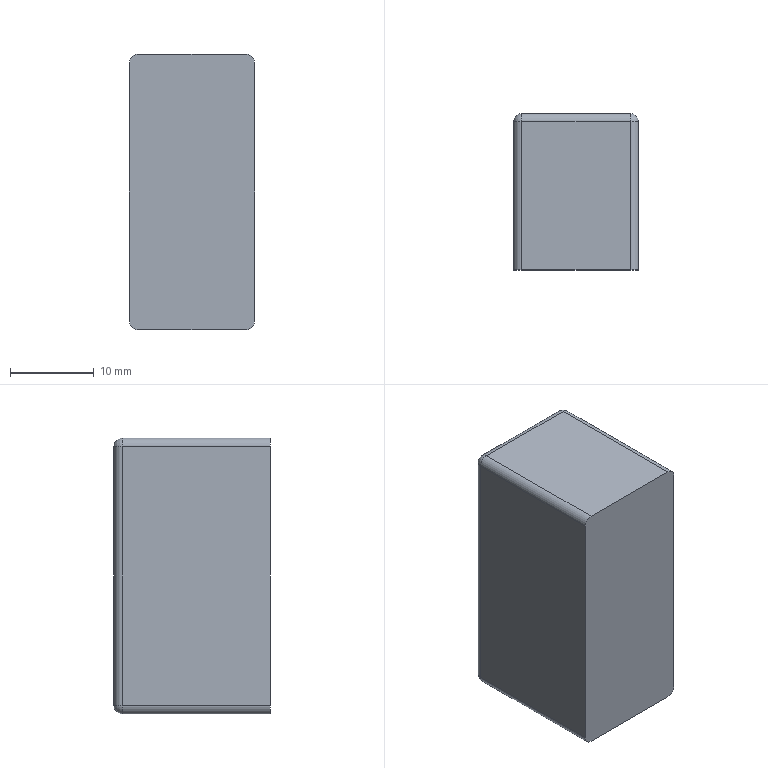Component | SolidWorks | StorageBox-1 | 1 solid | 23 faces | box 15 x 18.73 x 33 mm | volume 3493 mm3 | plane 11 | cylinder 8 | sphere 4 | commonest cylinder face diameters 2 x8
STEP:
#1=CARTESIAN_POINT('',(-0.8525,-3.531,8.395));
#2=VERTEX_POINT('',#1);
#3=CARTESIAN_POINT('',(-1.364,-3.531,8.395));
#4=VERTEX_POINT('',#3);
#5=CARTESIAN_POINT('',(-0.8131,-3.531,8.395));
#6=DIRECTION('',(-1.,-0.,0.));
#7=VECTOR('',#6,39.37);
#8=LINE('',#5,#7);
#9=EDGE_CURVE('',#2,#4,#8,.T.);
#10=ORIENTED_EDGE('',*,*,#9,.T.);
#11=CARTESIAN_POINT('',(-1.364,-4.229,8.395));
#12=VERTEX_POINT('',#11);
#13=CARTESIAN_POINT('',(-1.364,-4.229,8.395));
#14=DIRECTION('',(0.,-1.,0.));
#15=VECTOR('',#14,39.37);
#16=LINE('',#13,#15);
#17=EDGE_CURVE('',#4,#12,#16,.T.);
#18=ORIENTED_EDGE('',*,*,#17,.T.);
#19=CARTESIAN_POINT('',(-0.8525,-4.229,8.395));
#20=VERTEX_POINT('',#19);
#21=CARTESIAN_POINT('',(-0.8131,-4.229,8.395));
#22=DIRECTION('',(-1.,-0.,0.));
#23=VECTOR('',#22,39.37);
#24=LINE('',#21,#23);
#25=EDGE_CURVE('',#20,#12,#24,.T.);
#26=ORIENTED_EDGE('',*,*,#25,.F.);
#27=CARTESIAN_POINT('',(-0.8525,-4.229,8.395));
#28=DIRECTION('',(-0.,1.,-0.));
#29=VECTOR('',#28,39.37);
#30=LINE('',#27,#29);
#31=EDGE_CURVE('',#20,#2,#30,.T.);
#32=ORIENTED_EDGE('',*,*,#31,.T.);
#33=EDGE_LOOP('',(#10,#18,#26,#32));
#34=FACE_OUTER_BOUND('',#33,.T.);
#35=CARTESIAN_POINT('',(-0.8131,-4.229,8.395));
#36=DIRECTION('',(-0.,-0.,-1.));
#37=DIRECTION('',(-1.,-0.,0.));
#38=AXIS2_PLACEMENT_3D('',#35,#36,#37);
#39=PLANE('',#38);
#40=ADVANCED_FACE('',(#34),#39,.F.);
#41=CARTESIAN_POINT('',(-0.8525,-4.229,7.096));
#42=VERTEX_POINT('',#41);
#43=CARTESIAN_POINT('',(-1.364,-4.229,7.096));
#44=VERTEX_POINT('',#43);
#45=CARTESIAN_POINT('',(-0.8131,-4.229,7.096));
#46=DIRECTION('',(-1.,-0.,0.));
#47=VECTOR('',#46,39.37);
#48=LINE('',#45,#47);
#49=EDGE_CURVE('',#42,#44,#48,.T.);
#50=ORIENTED_EDGE('',*,*,#49,.F.);
#51=CARTESIAN_POINT('',(-0.8131,-4.229,7.136));
#52=VERTEX_POINT('',#51);
#53=CARTESIAN_POINT('',(-0.8525,-4.229,7.136));
#54=DIRECTION('',(0.,-1.,0.));
#55=DIRECTION('',(1.,0.,0.));
#56=AXIS2_PLACEMENT_3D('',#53,#54,#55);
#57=CIRCLE('',#56,0.03937);
#58=EDGE_CURVE('',#42,#52,#57,.T.);
#59=ORIENTED_EDGE('',*,*,#58,.T.);
#60=CARTESIAN_POINT('',(-0.8131,-4.229,8.356));
#61=VERTEX_POINT('',#60);
#62=CARTESIAN_POINT('',(-0.8131,-4.229,8.395));
#63=DIRECTION('',(-0.,-0.,-1.));
#64=VECTOR('',#63,39.37);
#65=LINE('',#62,#64);
#66=EDGE_CURVE('',#61,#52,#65,.T.);
#67=ORIENTED_EDGE('',*,*,#66,.F.);
#68=CARTESIAN_POINT('',(-0.8525,-4.229,8.356));
#69=DIRECTION('',(0.,-1.,0.));
#70=DIRECTION('',(1.,0.,0.));
#71=AXIS2_PLACEMENT_3D('',#68,#69,#70);
#72=CIRCLE('',#71,0.03937);
#73=EDGE_CURVE('',#61,#20,#72,.T.);
#74=ORIENTED_EDGE('',*,*,#73,.T.);
#75=ORIENTED_EDGE('',*,*,#25,.T.);
#76=CARTESIAN_POINT('',(-1.404,-4.229,8.356));
#77=VERTEX_POINT('',#76);
#78=CARTESIAN_POINT('',(-1.364,-4.229,8.356));
#79=DIRECTION('',(0.,-1.,0.));
#80=DIRECTION('',(1.,0.,0.));
#81=AXIS2_PLACEMENT_3D('',#78,#79,#80);
#82=CIRCLE('',#81,0.03937);
#83=EDGE_CURVE('',#12,#77,#82,.T.);
#84=ORIENTED_EDGE('',*,*,#83,.T.);
#85=CARTESIAN_POINT('',(-1.404,-4.229,7.136));
#86=VERTEX_POINT('',#85);
#87=CARTESIAN_POINT('',(-1.404,-4.229,8.395));
#88=DIRECTION('',(-0.,-0.,-1.));
#89=VECTOR('',#88,39.37);
#90=LINE('',#87,#89);
#91=EDGE_CURVE('',#77,#86,#90,.T.);
#92=ORIENTED_EDGE('',*,*,#91,.T.);
#93=CARTESIAN_POINT('',(-1.364,-4.229,7.136));
#94=DIRECTION('',(0.,-1.,0.));
#95=DIRECTION('',(1.,0.,0.));
#96=AXIS2_PLACEMENT_3D('',#93,#94,#95);
#97=CIRCLE('',#96,0.03937);
#98=EDGE_CURVE('',#86,#44,#97,.T.);
#99=ORIENTED_EDGE('',*,*,#98,.T.);
#100=EDGE_LOOP('',(#50,#59,#67,#74,#75,#84,#92,#99));
#101=FACE_OUTER_BOUND('',#100,.T.);
#102=CARTESIAN_POINT('',(-0.8131,-4.229,8.395));
#103=DIRECTION('',(-0.,1.,-0.));
#104=DIRECTION('',(1.,0.,-0.));
#105=AXIS2_PLACEMENT_3D('',#102,#103,#104);
#106=PLANE('',#105);
#107=ADVANCED_FACE('',(#101),#106,.F.);
#108=CARTESIAN_POINT('',(-1.364,-3.531,7.096));
#109=VERTEX_POINT('',#108);
#110=CARTESIAN_POINT('',(-0.8525,-3.531,7.096));
#111=VERTEX_POINT('',#110);
#112=CARTESIAN_POINT('',(-0.8131,-3.531,7.096));
#113=DIRECTION('',(1.,0.,-0.));
#114=VECTOR('',#113,39.37);
#115=LINE('',#112,#114);
#116=EDGE_CURVE('',#109,#111,#115,.T.);
#117=ORIENTED_EDGE('',*,*,#116,.T.);
#118=CARTESIAN_POINT('',(-0.8525,-4.229,7.096));
#119=DIRECTION('',(0.,-1.,0.));
#120=VECTOR('',#119,39.37);
#121=LINE('',#118,#120);
#122=EDGE_CURVE('',#111,#42,#121,.T.);
#123=ORIENTED_EDGE('',*,*,#122,.T.);
#124=ORIENTED_EDGE('',*,*,#49,.T.);
#125=CARTESIAN_POINT('',(-1.364,-3.531,7.096));
#126=DIRECTION('',(-0.,1.,-0.));
#127=VECTOR('',#126,39.37);
#128=LINE('',#125,#127);
#129=EDGE_CURVE('',#44,#109,#128,.T.);
#130=ORIENTED_EDGE('',*,*,#129,.T.);
#131=EDGE_LOOP('',(#117,#123,#124,#130));
#132=FACE_OUTER_BOUND('',#131,.T.);
#133=CARTESIAN_POINT('',(-0.8131,-4.229,7.096));
#134=DIRECTION('',(0.,0.,1.));
#135=DIRECTION('',(1.,0.,-0.));
#136=AXIS2_PLACEMENT_3D('',#133,#134,#135);
#137=PLANE('',#136);
#138=ADVANCED_FACE('',(#132),#137,.F.);
#139=CARTESIAN_POINT('',(-1.364,-3.492,8.356));
#140=VERTEX_POINT('',#139);
#141=CARTESIAN_POINT('',(-0.8525,-3.492,8.356));
#142=VERTEX_POINT('',#141);
#143=CARTESIAN_POINT('',(-0.8131,-3.492,8.356));
#144=DIRECTION('',(1.,0.,-0.));
#145=VECTOR('',#144,39.37);
#146=LINE('',#143,#145);
#147=EDGE_CURVE('',#140,#142,#146,.T.);
#148=ORIENTED_EDGE('',*,*,#147,.T.);
#149=CARTESIAN_POINT('',(-0.8525,-3.492,7.136));
#150=VERTEX_POINT('',#149);
#151=CARTESIAN_POINT('',(-0.8525,-3.492,8.395));
#152=DIRECTION('',(-0.,-0.,-1.));
#153=VECTOR('',#152,39.37);
#154=LINE('',#151,#153);
#155=EDGE_CURVE('',#142,#150,#154,.T.);
#156=ORIENTED_EDGE('',*,*,#155,.T.);
#157=CARTESIAN_POINT('',(-1.364,-3.492,7.136));
#158=VERTEX_POINT('',#157);
#159=CARTESIAN_POINT('',(-0.8131,-3.492,7.136));
#160=DIRECTION('',(-1.,-0.,0.));
#161=VECTOR('',#160,39.37);
#162=LINE('',#159,#161);
#163=EDGE_CURVE('',#150,#158,#162,.T.);
#164=ORIENTED_EDGE('',*,*,#163,.T.);
#165=CARTESIAN_POINT('',(-1.364,-3.492,8.395));
#166=DIRECTION('',(0.,0.,1.));
#167=VECTOR('',#166,39.37);
#168=LINE('',#165,#167);
#169=EDGE_CURVE('',#158,#140,#168,.T.);
#170=ORIENTED_EDGE('',*,*,#169,.T.);
#171=EDGE_LOOP('',(#148,#156,#164,#170));
#172=FACE_OUTER_BOUND('',#171,.T.);
#173=CARTESIAN_POINT('',(-1.325,-3.492,7.175));
#174=VERTEX_POINT('',#173);
#175=CARTESIAN_POINT('',(-1.325,-3.492,8.317));
#176=VERTEX_POINT('',#175);
#177=CARTESIAN_POINT('',(-1.325,-3.492,7.175));
#178=DIRECTION('',(0.,0.,1.));
#179=VECTOR('',#178,39.37);
#180=LINE('',#177,#179);
#181=EDGE_CURVE('',#174,#176,#180,.T.);
#182=ORIENTED_EDGE('',*,*,#181,.F.);
#183=CARTESIAN_POINT('',(-0.8919,-3.492,7.175));
#184=VERTEX_POINT('',#183);
#185=CARTESIAN_POINT('',(-0.8919,-3.492,7.175));
#186=DIRECTION('',(-1.,-0.,0.));
#187=VECTOR('',#186,39.37);
#188=LINE('',#185,#187);
#189=EDGE_CURVE('',#184,#174,#188,.T.);
#190=ORIENTED_EDGE('',*,*,#189,.F.);
#191=CARTESIAN_POINT('',(-0.8919,-3.492,8.317));
#192=VERTEX_POINT('',#191);
#193=CARTESIAN_POINT('',(-0.8919,-3.492,8.317));
#194=DIRECTION('',(-0.,-0.,-1.));
#195=VECTOR('',#194,39.37);
#196=LINE('',#193,#195);
#197=EDGE_CURVE('',#192,#184,#196,.T.);
#198=ORIENTED_EDGE('',*,*,#197,.F.);
#199=CARTESIAN_POINT('',(-1.325,-3.492,8.317));
#200=DIRECTION('',(1.,0.,-0.));
#201=VECTOR('',#200,39.37);
#202=LINE('',#199,#201);
#203=EDGE_CURVE('',#176,#192,#202,.T.);
#204=ORIENTED_EDGE('',*,*,#203,.F.);
#205=EDGE_LOOP('',(#182,#190,#198,#204));
#206=FACE_BOUND('',#205,.T.);
#207=CARTESIAN_POINT('',(-0.8131,-3.492,8.395));
#208=DIRECTION('',(0.,-1.,0.));
#209=DIRECTION('',(-1.,-0.,0.));
#210=AXIS2_PLACEMENT_3D('',#207,#208,#209);
#211=PLANE('',#210);
#212=ADVANCED_FACE('',(#172,#206),#211,.F.);
#213=ORIENTED_EDGE('',*,*,#66,.T.);
#214=CARTESIAN_POINT('',(-0.8131,-3.531,7.136));
#215=VERTEX_POINT('',#214);
#216=CARTESIAN_POINT('',(-0.8131,-4.229,7.136));
#217=DIRECTION('',(-0.,1.,-0.));
#218=VECTOR('',#217,39.37);
#219=LINE('',#216,#218);
#220=EDGE_CURVE('',#52,#215,#219,.T.);
#221=ORIENTED_EDGE('',*,*,#220,.T.);
#222=CARTESIAN_POINT('',(-0.8131,-3.531,8.356));
#223=VERTEX_POINT('',#222);
#224=CARTESIAN_POINT('',(-0.8131,-3.531,8.395));
#225=DIRECTION('',(0.,0.,1.));
#226=VECTOR('',#225,39.37);
#227=LINE('',#224,#226);
#228=EDGE_CURVE('',#215,#223,#227,.T.);
#229=ORIENTED_EDGE('',*,*,#228,.T.);
#230=CARTESIAN_POINT('',(-0.8131,-4.229,8.356));
#231=DIRECTION('',(0.,-1.,0.));
#232=VECTOR('',#231,39.37);
#233=LINE('',#230,#232);
#234=EDGE_CURVE('',#223,#61,#233,.T.);
#235=ORIENTED_EDGE('',*,*,#234,.T.);
#236=EDGE_LOOP('',(#213,#221,#229,#235));
#237=FACE_OUTER_BOUND('',#236,.T.);
#238=CARTESIAN_POINT('',(-0.8131,-4.229,8.395));
#239=DIRECTION('',(-1.,-0.,0.));
#240=DIRECTION('',(0.,0.,1.));
#241=AXIS2_PLACEMENT_3D('',#238,#239,#240);
#242=PLANE('',#241);
#243=ADVANCED_FACE('',(#237),#242,.F.);
#244=CARTESIAN_POINT('',(-1.404,-3.531,8.356));
#245=VERTEX_POINT('',#244);
#246=CARTESIAN_POINT('',(-1.404,-3.531,7.136));
#247=VERTEX_POINT('',#246);
#248=CARTESIAN_POINT('',(-1.404,-3.531,7.096));
#249=DIRECTION('',(-0.,-0.,-1.));
#250=VECTOR('',#249,39.37);
#251=LINE('',#248,#250);
#252=EDGE_CURVE('',#245,#247,#251,.T.);
#253=ORIENTED_EDGE('',*,*,#252,.T.);
#254=CARTESIAN_POINT('',(-1.404,-4.229,7.136));
#255=DIRECTION('',(0.,-1.,0.));
#256=VECTOR('',#255,39.37);
#257=LINE('',#254,#256);
#258=EDGE_CURVE('',#247,#86,#257,.T.);
#259=ORIENTED_EDGE('',*,*,#258,.T.);
#260=ORIENTED_EDGE('',*,*,#91,.F.);
#261=CARTESIAN_POINT('',(-1.404,-3.531,8.356));
#262=DIRECTION('',(-0.,1.,-0.));
#263=VECTOR('',#262,39.37);
#264=LINE('',#261,#263);
#265=EDGE_CURVE('',#77,#245,#264,.T.);
#266=ORIENTED_EDGE('',*,*,#265,.T.);
#267=EDGE_LOOP('',(#253,#259,#260,#266));
#268=FACE_OUTER_BOUND('',#267,.T.);
#269=CARTESIAN_POINT('',(-1.404,-4.229,8.395));
#270=DIRECTION('',(-1.,-0.,0.));
#271=DIRECTION('',(0.,0.,1.));
#272=AXIS2_PLACEMENT_3D('',#269,#270,#271);
#273=PLANE('',#272);
#274=ADVANCED_FACE('',(#268),#273,.T.);
#275=ORIENTED_EDGE('',*,*,#189,.T.);
#276=CARTESIAN_POINT('',(-1.325,-4.2,7.175));
#277=VERTEX_POINT('',#276);
#278=CARTESIAN_POINT('',(-1.325,-4.2,7.175));
#279=DIRECTION('',(-0.,1.,-0.));
#280=VECTOR('',#279,39.37);
#281=LINE('',#278,#280);
#282=EDGE_CURVE('',#277,#174,#281,.T.);
#283=ORIENTED_EDGE('',*,*,#282,.F.);
#284=CARTESIAN_POINT('',(-0.8919,-4.2,7.175));
#285=VERTEX_POINT('',#284);
#286=CARTESIAN_POINT('',(-0.8919,-4.2,7.175));
#287=DIRECTION('',(-1.,-0.,0.));
#288=VECTOR('',#287,39.37);
#289=LINE('',#286,#288);
#290=EDGE_CURVE('',#285,#277,#289,.T.);
#291=ORIENTED_EDGE('',*,*,#290,.F.);
#292=CARTESIAN_POINT('',(-0.8919,-4.2,7.175));
#293=DIRECTION('',(-0.,1.,-0.));
#294=VECTOR('',#293,39.37);
#295=LINE('',#292,#294);
#296=EDGE_CURVE('',#285,#184,#295,.T.);
#297=ORIENTED_EDGE('',*,*,#296,.T.);
#298=EDGE_LOOP('',(#275,#283,#291,#297));
#299=FACE_OUTER_BOUND('',#298,.T.);
#300=CARTESIAN_POINT('',(-0.8919,-4.2,7.175));
#301=DIRECTION('',(-0.,-0.,-1.));
#302=DIRECTION('',(-1.,-0.,0.));
#303=AXIS2_PLACEMENT_3D('',#300,#301,#302);
#304=PLANE('',#303);
#305=ADVANCED_FACE('',(#299),#304,.F.);
#306=ORIENTED_EDGE('',*,*,#197,.T.);
#307=ORIENTED_EDGE('',*,*,#296,.F.);
#308=CARTESIAN_POINT('',(-0.8919,-4.2,8.317));
#309=VERTEX_POINT('',#308);
#310=CARTESIAN_POINT('',(-0.8919,-4.2,8.317));
#311=DIRECTION('',(-0.,-0.,-1.));
#312=VECTOR('',#311,39.37);
#313=LINE('',#310,#312);
#314=EDGE_CURVE('',#309,#285,#313,.T.);
#315=ORIENTED_EDGE('',*,*,#314,.F.);
#316=CARTESIAN_POINT('',(-0.8919,-4.2,8.317));
#317=DIRECTION('',(-0.,1.,-0.));
#318=VECTOR('',#317,39.37);
#319=LINE('',#316,#318);
#320=EDGE_CURVE('',#309,#192,#319,.T.);
#321=ORIENTED_EDGE('',*,*,#320,.T.);
#322=EDGE_LOOP('',(#306,#307,#315,#321));
#323=FACE_OUTER_BOUND('',#322,.T.);
#324=CARTESIAN_POINT('',(-0.8919,-4.2,8.317));
#325=DIRECTION('',(1.,0.,-0.));
#326=DIRECTION('',(-0.,-0.,-1.));
#327=AXIS2_PLACEMENT_3D('',#324,#325,#326);
#328=PLANE('',#327);
#329=ADVANCED_FACE('',(#323),#328,.F.);
#330=ORIENTED_EDGE('',*,*,#203,.T.);
#331=ORIENTED_EDGE('',*,*,#320,.F.);
#332=CARTESIAN_POINT('',(-1.325,-4.2,8.317));
#333=VERTEX_POINT('',#332);
#334=CARTESIAN_POINT('',(-1.325,-4.2,8.317));
#335=DIRECTION('',(1.,0.,-0.));
#336=VECTOR('',#335,39.37);
#337=LINE('',#334,#336);
#338=EDGE_CURVE('',#333,#309,#337,.T.);
#339=ORIENTED_EDGE('',*,*,#338,.F.);
#340=CARTESIAN_POINT('',(-1.325,-4.2,8.317));
#341=DIRECTION('',(-0.,1.,-0.));
#342=VECTOR('',#341,39.37);
#343=LINE('',#340,#342);
#344=EDGE_CURVE('',#333,#176,#343,.T.);
#345=ORIENTED_EDGE('',*,*,#344,.T.);
#346=EDGE_LOOP('',(#330,#331,#339,#345));
#347=FACE_OUTER_BOUND('',#346,.T.);
#348=CARTESIAN_POINT('',(-1.325,-4.2,8.317));
#349=DIRECTION('',(0.,0.,1.));
#350=DIRECTION('',(1.,0.,-0.));
#351=AXIS2_PLACEMENT_3D('',#348,#349,#350);
#352=PLANE('',#351);
#353=ADVANCED_FACE('',(#347),#352,.F.);
#354=ORIENTED_EDGE('',*,*,#181,.T.);
#355=ORIENTED_EDGE('',*,*,#344,.F.);
#356=CARTESIAN_POINT('',(-1.325,-4.2,7.175));
#357=DIRECTION('',(0.,0.,1.));
#358=VECTOR('',#357,39.37);
#359=LINE('',#356,#358);
#360=EDGE_CURVE('',#277,#333,#359,.T.);
#361=ORIENTED_EDGE('',*,*,#360,.F.);
#362=ORIENTED_EDGE('',*,*,#282,.T.);
#363=EDGE_LOOP('',(#354,#355,#361,#362));
#364=FACE_OUTER_BOUND('',#363,.T.);
#365=CARTESIAN_POINT('',(-1.325,-4.2,7.175));
#366=DIRECTION('',(-1.,-0.,0.));
#367=DIRECTION('',(0.,0.,1.));
#368=AXIS2_PLACEMENT_3D('',#365,#366,#367);
#369=PLANE('',#368);
#370=ADVANCED_FACE('',(#364),#369,.F.);
#371=ORIENTED_EDGE('',*,*,#290,.T.);
#372=ORIENTED_EDGE('',*,*,#360,.T.);
#373=ORIENTED_EDGE('',*,*,#338,.T.);
#374=ORIENTED_EDGE('',*,*,#314,.T.);
#375=EDGE_LOOP('',(#371,#372,#373,#374));
#376=FACE_OUTER_BOUND('',#375,.T.);
#377=CARTESIAN_POINT('',(-1.404,-4.2,8.395));
#378=DIRECTION('',(-0.,1.,-0.));
#379=DIRECTION('',(1.,0.,-0.));
#380=AXIS2_PLACEMENT_3D('',#377,#378,#379);
#381=PLANE('',#380);
#382=ADVANCED_FACE('',(#376),#381,.T.);
#383=ORIENTED_EDGE('',*,*,#169,.F.);
#384=CARTESIAN_POINT('',(-1.364,-3.531,7.136));
#385=DIRECTION('',(0.,0.,1.));
#386=DIRECTION('',(-1.,0.,0.));
#387=AXIS2_PLACEMENT_3D('',#384,#385,#386);
#388=CIRCLE('',#387,0.03937);
#389=EDGE_CURVE('',#158,#247,#388,.T.);
#390=ORIENTED_EDGE('',*,*,#389,.T.);
#391=ORIENTED_EDGE('',*,*,#252,.F.);
#392=CARTESIAN_POINT('',(-1.364,-3.531,8.356));
#393=DIRECTION('',(-0.,-0.,-1.));
#394=DIRECTION('',(-1.,0.,0.));
#395=AXIS2_PLACEMENT_3D('',#392,#393,#394);
#396=CIRCLE('',#395,0.03937);
#397=EDGE_CURVE('',#245,#140,#396,.T.);
#398=ORIENTED_EDGE('',*,*,#397,.T.);
#399=EDGE_LOOP('',(#383,#390,#391,#398));
#400=FACE_OUTER_BOUND('',#399,.T.);
#401=CARTESIAN_POINT('',(-1.364,-3.531,8.395));
#402=DIRECTION('',(-0.,-0.,-1.));
#403=DIRECTION('',(-1.,0.,0.));
#404=AXIS2_PLACEMENT_3D('',#401,#402,#403);
#405=CYLINDRICAL_SURFACE('',#404,0.03937);
#406=ADVANCED_FACE('',(#400),#405,.T.);
#407=ORIENTED_EDGE('',*,*,#163,.F.);
#408=CARTESIAN_POINT('',(-0.8525,-3.531,7.136));
#409=DIRECTION('',(-1.,-0.,0.));
#410=DIRECTION('',(0.,0.,1.));
#411=AXIS2_PLACEMENT_3D('',#408,#409,#410);
#412=CIRCLE('',#411,0.03937);
#413=EDGE_CURVE('',#150,#111,#412,.T.);
#414=ORIENTED_EDGE('',*,*,#413,.T.);
#415=ORIENTED_EDGE('',*,*,#116,.F.);
#416=CARTESIAN_POINT('',(-1.364,-3.531,7.136));
#417=DIRECTION('',(1.,0.,-0.));
#418=DIRECTION('',(0.,0.,1.));
#419=AXIS2_PLACEMENT_3D('',#416,#417,#418);
#420=CIRCLE('',#419,0.03937);
#421=EDGE_CURVE('',#109,#158,#420,.T.);
#422=ORIENTED_EDGE('',*,*,#421,.T.);
#423=EDGE_LOOP('',(#407,#414,#415,#422));
#424=FACE_OUTER_BOUND('',#423,.T.);
#425=CARTESIAN_POINT('',(-0.8131,-3.531,7.136));
#426=DIRECTION('',(-1.,-0.,0.));
#427=DIRECTION('',(0.,0.,1.));
#428=AXIS2_PLACEMENT_3D('',#425,#426,#427);
#429=CYLINDRICAL_SURFACE('',#428,0.03937);
#430=ADVANCED_FACE('',(#424),#429,.T.);
#431=ORIENTED_EDGE('',*,*,#147,.F.);
#432=CARTESIAN_POINT('',(-1.364,-3.531,8.356));
#433=DIRECTION('',(1.,0.,-0.));
#434=DIRECTION('',(0.,0.,1.));
#435=AXIS2_PLACEMENT_3D('',#432,#433,#434);
#436=CIRCLE('',#435,0.03937);
#437=EDGE_CURVE('',#140,#4,#436,.T.);
#438=ORIENTED_EDGE('',*,*,#437,.T.);
#439=ORIENTED_EDGE('',*,*,#9,.F.);
#440=CARTESIAN_POINT('',(-0.8525,-3.531,8.356));
#441=DIRECTION('',(-1.,-0.,0.));
#442=DIRECTION('',(0.,0.,1.));
#443=AXIS2_PLACEMENT_3D('',#440,#441,#442);
#444=CIRCLE('',#443,0.03937);
#445=EDGE_CURVE('',#2,#142,#444,.T.);
#446=ORIENTED_EDGE('',*,*,#445,.T.);
#447=EDGE_LOOP('',(#431,#438,#439,#446));
#448=FACE_OUTER_BOUND('',#447,.T.);
#449=CARTESIAN_POINT('',(-0.8131,-3.531,8.356));
#450=DIRECTION('',(-1.,-0.,0.));
#451=DIRECTION('',(0.,0.,1.));
#452=AXIS2_PLACEMENT_3D('',#449,#450,#451);
#453=CYLINDRICAL_SURFACE('',#452,0.03937);
#454=ADVANCED_FACE('',(#448),#453,.T.);
#455=ORIENTED_EDGE('',*,*,#228,.F.);
#456=CARTESIAN_POINT('',(-0.8525,-3.531,7.136));
#457=DIRECTION('',(0.,0.,1.));
#458=DIRECTION('',(1.,0.,0.));
#459=AXIS2_PLACEMENT_3D('',#456,#457,#458);
#460=CIRCLE('',#459,0.03937);
#461=EDGE_CURVE('',#215,#150,#460,.T.);
#462=ORIENTED_EDGE('',*,*,#461,.T.);
#463=ORIENTED_EDGE('',*,*,#155,.F.);
#464=CARTESIAN_POINT('',(-0.8525,-3.531,8.356));
#465=DIRECTION('',(-0.,-0.,-1.));
#466=DIRECTION('',(1.,0.,0.));
#467=AXIS2_PLACEMENT_3D('',#464,#465,#466);
#468=CIRCLE('',#467,0.03937);
#469=EDGE_CURVE('',#142,#223,#468,.T.);
#470=ORIENTED_EDGE('',*,*,#469,.T.);
#471=EDGE_LOOP('',(#455,#462,#463,#470));
#472=FACE_OUTER_BOUND('',#471,.T.);
#473=CARTESIAN_POINT('',(-0.8525,-3.531,8.395));
#474=DIRECTION('',(0.,0.,1.));
#475=DIRECTION('',(1.,0.,0.));
#476=AXIS2_PLACEMENT_3D('',#473,#474,#475);
#477=CYLINDRICAL_SURFACE('',#476,0.03937);
#478=ADVANCED_FACE('',(#472),#477,.T.);
#479=ORIENTED_EDGE('',*,*,#58,.F.);
#480=ORIENTED_EDGE('',*,*,#122,.F.);
#481=CARTESIAN_POINT('',(-0.8525,-3.531,7.136));
#482=DIRECTION('',(-0.,1.,-0.));
#483=DIRECTION('',(1.,0.,0.));
#484=AXIS2_PLACEMENT_3D('',#481,#482,#483);
#485=CIRCLE('',#484,0.03937);
#486=EDGE_CURVE('',#215,#111,#485,.T.);
#487=ORIENTED_EDGE('',*,*,#486,.F.);
#488=ORIENTED_EDGE('',*,*,#220,.F.);
#489=EDGE_LOOP('',(#479,#480,#487,#488));
#490=FACE_OUTER_BOUND('',#489,.T.);
#491=CARTESIAN_POINT('',(-0.8525,-4.229,7.136));
#492=DIRECTION('',(-0.,1.,-0.));
#493=DIRECTION('',(1.,0.,0.));
#494=AXIS2_PLACEMENT_3D('',#491,#492,#493);
#495=CYLINDRICAL_SURFACE('',#494,0.03937);
#496=ADVANCED_FACE('',(#490),#495,.T.);
#497=ORIENTED_EDGE('',*,*,#486,.T.);
#498=ORIENTED_EDGE('',*,*,#413,.F.);
#499=ORIENTED_EDGE('',*,*,#461,.F.);
#500=EDGE_LOOP('',(#497,#498,#499));
#501=FACE_OUTER_BOUND('',#500,.T.);
#502=CARTESIAN_POINT('',(-0.8525,-3.531,7.136));
#503=DIRECTION('',(-0.,1.,0.));
#504=DIRECTION('',(0.,0.,-1.));
#505=AXIS2_PLACEMENT_3D('',#502,#503,#504);
#506=SPHERICAL_SURFACE('',#505,0.03937);
#507=ADVANCED_FACE('',(#501),#506,.T.);
#508=ORIENTED_EDGE('',*,*,#98,.F.);
#509=ORIENTED_EDGE('',*,*,#258,.F.);
#510=CARTESIAN_POINT('',(-1.364,-3.531,7.136));
#511=DIRECTION('',(-0.,1.,-0.));
#512=DIRECTION('',(1.,0.,0.));
#513=AXIS2_PLACEMENT_3D('',#510,#511,#512);
#514=CIRCLE('',#513,0.03937);
#515=EDGE_CURVE('',#109,#247,#514,.T.);
#516=ORIENTED_EDGE('',*,*,#515,.F.);
#517=ORIENTED_EDGE('',*,*,#129,.F.);
#518=EDGE_LOOP('',(#508,#509,#516,#517));
#519=FACE_OUTER_BOUND('',#518,.T.);
#520=CARTESIAN_POINT('',(-1.364,-4.229,7.136));
#521=DIRECTION('',(0.,-1.,0.));
#522=DIRECTION('',(-1.,0.,0.));
#523=AXIS2_PLACEMENT_3D('',#520,#521,#522);
#524=CYLINDRICAL_SURFACE('',#523,0.03937);
#525=ADVANCED_FACE('',(#519),#524,.T.);
#526=ORIENTED_EDGE('',*,*,#515,.T.);
#527=ORIENTED_EDGE('',*,*,#389,.F.);
#528=ORIENTED_EDGE('',*,*,#421,.F.);
#529=EDGE_LOOP('',(#526,#527,#528));
#530=FACE_OUTER_BOUND('',#529,.T.);
#531=CARTESIAN_POINT('',(-1.364,-3.531,7.136));
#532=DIRECTION('',(-0.,1.,0.));
#533=DIRECTION('',(0.,0.,-1.));
#534=AXIS2_PLACEMENT_3D('',#531,#532,#533);
#535=SPHERICAL_SURFACE('',#534,0.03937);
#536=ADVANCED_FACE('',(#530),#535,.T.);
#537=ORIENTED_EDGE('',*,*,#83,.F.);
#538=ORIENTED_EDGE('',*,*,#17,.F.);
#539=CARTESIAN_POINT('',(-1.364,-3.531,8.356));
#540=DIRECTION('',(-0.,1.,-0.));
#541=DIRECTION('',(1.,0.,0.));
#542=AXIS2_PLACEMENT_3D('',#539,#540,#541);
#543=CIRCLE('',#542,0.03937);
#544=EDGE_CURVE('',#245,#4,#543,.T.);
#545=ORIENTED_EDGE('',*,*,#544,.F.);
#546=ORIENTED_EDGE('',*,*,#265,.F.);
#547=EDGE_LOOP('',(#537,#538,#545,#546));
#548=FACE_OUTER_BOUND('',#547,.T.);
#549=CARTESIAN_POINT('',(-1.364,-4.229,8.356));
#550=DIRECTION('',(-0.,1.,-0.));
#551=DIRECTION('',(1.,0.,0.));
#552=AXIS2_PLACEMENT_3D('',#549,#550,#551);
#553=CYLINDRICAL_SURFACE('',#552,0.03937);
#554=ADVANCED_FACE('',(#548),#553,.T.);
#555=ORIENTED_EDGE('',*,*,#437,.F.);
#556=ORIENTED_EDGE('',*,*,#397,.F.);
#557=ORIENTED_EDGE('',*,*,#544,.T.);
#558=EDGE_LOOP('',(#555,#556,#557));
#559=FACE_OUTER_BOUND('',#558,.T.);
#560=CARTESIAN_POINT('',(-1.364,-3.531,8.356));
#561=DIRECTION('',(-0.,1.,0.));
#562=DIRECTION('',(0.,0.,-1.));
#563=AXIS2_PLACEMENT_3D('',#560,#561,#562);
#564=SPHERICAL_SURFACE('',#563,0.03937);
#565=ADVANCED_FACE('',(#559),#564,.T.);
#566=ORIENTED_EDGE('',*,*,#73,.F.);
#567=ORIENTED_EDGE('',*,*,#234,.F.);
#568=CARTESIAN_POINT('',(-0.8525,-3.531,8.356));
#569=DIRECTION('',(-0.,1.,-0.));
#570=DIRECTION('',(1.,0.,0.));
#571=AXIS2_PLACEMENT_3D('',#568,#569,#570);
#572=CIRCLE('',#571,0.03937);
#573=EDGE_CURVE('',#2,#223,#572,.T.);
#574=ORIENTED_EDGE('',*,*,#573,.F.);
#575=ORIENTED_EDGE('',*,*,#31,.F.);
#576=EDGE_LOOP('',(#566,#567,#574,#575));
#577=FACE_OUTER_BOUND('',#576,.T.);
#578=CARTESIAN_POINT('',(-0.8525,-4.229,8.356));
#579=DIRECTION('',(0.,-1.,0.));
#580=DIRECTION('',(-1.,0.,0.));
#581=AXIS2_PLACEMENT_3D('',#578,#579,#580);
#582=CYLINDRICAL_SURFACE('',#581,0.03937);
#583=ADVANCED_FACE('',(#577),#582,.T.);
#584=ORIENTED_EDGE('',*,*,#469,.F.);
#585=ORIENTED_EDGE('',*,*,#445,.F.);
#586=ORIENTED_EDGE('',*,*,#573,.T.);
#587=EDGE_LOOP('',(#584,#585,#586));
#588=FACE_OUTER_BOUND('',#587,.T.);
#589=CARTESIAN_POINT('',(-0.8525,-3.531,8.356));
#590=DIRECTION('',(-0.,1.,0.));
#591=DIRECTION('',(0.,0.,-1.));
#592=AXIS2_PLACEMENT_3D('',#589,#590,#591);
#593=SPHERICAL_SURFACE('',#592,0.03937);
#594=ADVANCED_FACE('',(#588),#593,.T.);
#595=CLOSED_SHELL('',(#40,#107,#138,#212,#243,#274,#305,#329,#353,#370,#382,#406,#430,#454,#478,#496,#507,#525,#536,#554,#565,#583,#594));
#596=MANIFOLD_SOLID_BREP('',#595);
#597=CARTESIAN_POINT('',(0.,0.,0.));
#598=DIRECTION('',(0.,0.,1.));
#599=DIRECTION('',(1.,0.,0.));
#600=AXIS2_PLACEMENT_3D('',#597,#598,#599);
#601=(LENGTH_UNIT()NAMED_UNIT(*)SI_UNIT($,.METRE.));
#602=LENGTH_MEASURE_WITH_UNIT(LENGTH_MEASURE(0.0254),#601);
#603=DIMENSIONAL_EXPONENTS(1.,0.,0.,0.,0.,0.,0.);
#604=(CONVERSION_BASED_UNIT('',#602)LENGTH_UNIT()NAMED_UNIT(#603));
#605=UNCERTAINTY_MEASURE_WITH_UNIT(LENGTH_MEASURE(0.00001),#604,'','');
#606=(NAMED_UNIT(*)PLANE_ANGLE_UNIT()SI_UNIT($,.RADIAN.));
#607=(NAMED_UNIT(*)SI_UNIT($,.STERADIAN.)SOLID_ANGLE_UNIT());
#608=(GEOMETRIC_REPRESENTATION_CONTEXT(3)GLOBAL_UNCERTAINTY_ASSIGNED_CONTEXT((#605))GLOBAL_UNIT_ASSIGNED_CONTEXT((#604,#606,#607))REPRESENTATION_CONTEXT('',''));
#609=ADVANCED_BREP_SHAPE_REPRESENTATION('',(#596,#600),#608);
#610=COLOUR_RGB('',0.7922,0.8196,0.9333);
#611=FILL_AREA_STYLE_COLOUR('',#610);
#612=FILL_AREA_STYLE('',(#611));
#613=SURFACE_STYLE_FILL_AREA(#612);
#614=SURFACE_SIDE_STYLE('',(#613));
#615=SURFACE_STYLE_USAGE(.BOTH.,#614);
#616=PRESENTATION_STYLE_ASSIGNMENT((#615));
#617=STYLED_ITEM('',(#616),#596);
#618=(LENGTH_UNIT()NAMED_UNIT(*)SI_UNIT($,.METRE.));
#619=LENGTH_MEASURE_WITH_UNIT(LENGTH_MEASURE(0.0254),#618);
#620=DIMENSIONAL_EXPONENTS(1.,0.,0.,0.,0.,0.,0.);
#621=(CONVERSION_BASED_UNIT('',#619)LENGTH_UNIT()NAMED_UNIT(#620));
#622=UNCERTAINTY_MEASURE_WITH_UNIT(LENGTH_MEASURE(0.00001),#621,'','');
#623=(NAMED_UNIT(*)PLANE_ANGLE_UNIT()SI_UNIT($,.RADIAN.));
#624=(NAMED_UNIT(*)SI_UNIT($,.STERADIAN.)SOLID_ANGLE_UNIT());
#625=(GEOMETRIC_REPRESENTATION_CONTEXT(3)GLOBAL_UNCERTAINTY_ASSIGNED_CONTEXT((#622))GLOBAL_UNIT_ASSIGNED_CONTEXT((#621,#623,#624))REPRESENTATION_CONTEXT('',''));
#626=MECHANICAL_DESIGN_GEOMETRIC_PRESENTATION_REPRESENTATION('',(#617),#625);
#627=PRESENTATION_LAYER_ASSIGNMENT('','',(#617));